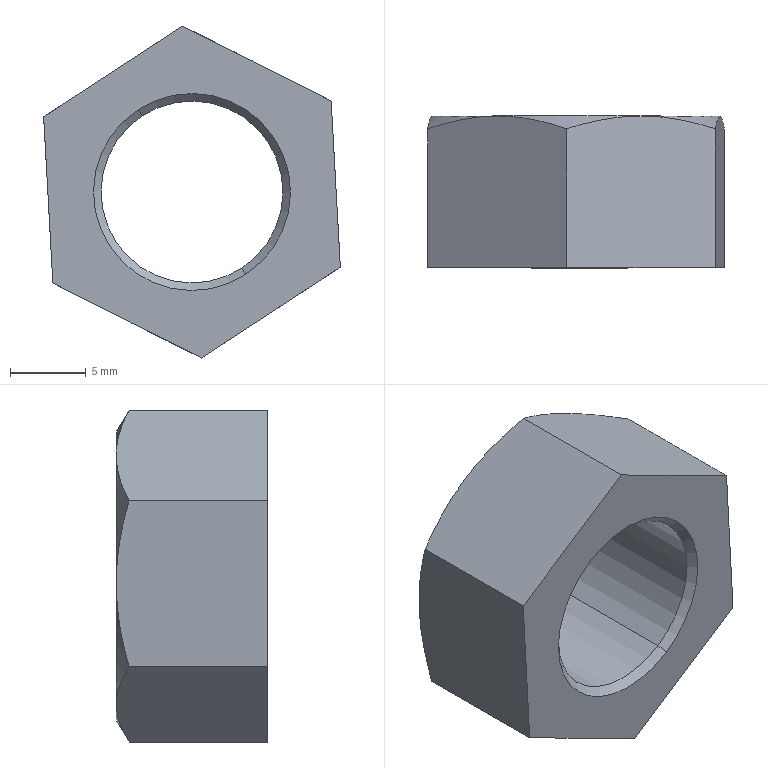Component | SolidWorks | TBK51-M12-4 | 1 solid | 20 faces | box 19.58 x 10 x 21.91 mm | volume 1978 mm3 | cone 10 | plane 8 | cylinder 2 | commonest cylinder face diameters 12 x2
STEP:
#1=CARTESIAN_POINT('',(-1.368,2.313,8.835));
#2=VERTEX_POINT('',#1);
#3=CARTESIAN_POINT('',(-1.627,2.313,9.231));
#4=VERTEX_POINT('',#3);
#5=CARTESIAN_POINT('',(-1.497,2.313,9.033));
#6=DIRECTION('',(0.,1.,-0.));
#7=DIRECTION('',(-0.5469,0.,0.8372));
#8=AXIS2_PLACEMENT_3D('',#5,#6,#7);
#9=CIRCLE('',#8,0.2362);
#10=EDGE_CURVE('',#2,#4,#9,.T.);
#11=ORIENTED_EDGE('',*,*,#10,.T.);
#12=CARTESIAN_POINT('',(-1.637,2.293,9.247));
#13=VERTEX_POINT('',#12);
#14=CARTESIAN_POINT('',(-1.627,2.313,9.231));
#15=DIRECTION('',(-0.3867,-0.7071,0.592));
#16=VECTOR('',#15,39.37);
#17=LINE('',#14,#16);
#18=EDGE_CURVE('',#4,#13,#17,.T.);
#19=ORIENTED_EDGE('',*,*,#18,.T.);
#20=CARTESIAN_POINT('',(-1.358,2.293,8.819));
#21=VERTEX_POINT('',#20);
#22=CARTESIAN_POINT('',(-1.497,2.293,9.033));
#23=DIRECTION('',(0.,1.,-0.));
#24=DIRECTION('',(-0.5469,0.,0.8372));
#25=AXIS2_PLACEMENT_3D('',#22,#23,#24);
#26=CIRCLE('',#25,0.2559);
#27=EDGE_CURVE('',#21,#13,#26,.T.);
#28=ORIENTED_EDGE('',*,*,#27,.F.);
#29=CARTESIAN_POINT('',(-1.368,2.313,8.835));
#30=DIRECTION('',(0.3867,-0.7071,-0.592));
#31=VECTOR('',#30,39.37);
#32=LINE('',#29,#31);
#33=EDGE_CURVE('',#2,#21,#32,.T.);
#34=ORIENTED_EDGE('',*,*,#33,.F.);
#35=EDGE_LOOP('',(#11,#19,#28,#34));
#36=FACE_OUTER_BOUND('',#35,.T.);
#37=CARTESIAN_POINT('',(-1.497,2.313,9.033));
#38=DIRECTION('',(-0.,-1.,0.));
#39=DIRECTION('',(0.5469,-0.,-0.8372));
#40=AXIS2_PLACEMENT_3D('',#37,#38,#39);
#41=CONICAL_SURFACE('',#40,0.2362,0.7854);
#42=ADVANCED_FACE('',(#36),#41,.F.);
#43=ORIENTED_EDGE('',*,*,#10,.F.);
#44=CARTESIAN_POINT('',(-1.368,2.667,8.835));
#45=VERTEX_POINT('',#44);
#46=CARTESIAN_POINT('',(-1.368,0.7185,8.835));
#47=DIRECTION('',(0.,1.,-0.));
#48=VECTOR('',#47,39.37);
#49=LINE('',#46,#48);
#50=EDGE_CURVE('',#2,#45,#49,.T.);
#51=ORIENTED_EDGE('',*,*,#50,.T.);
#52=CARTESIAN_POINT('',(-1.627,2.667,9.231));
#53=VERTEX_POINT('',#52);
#54=CARTESIAN_POINT('',(-1.497,2.667,9.033));
#55=DIRECTION('',(0.,1.,-0.));
#56=DIRECTION('',(-0.5469,0.,0.8372));
#57=AXIS2_PLACEMENT_3D('',#54,#55,#56);
#58=CIRCLE('',#57,0.2362);
#59=EDGE_CURVE('',#45,#53,#58,.T.);
#60=ORIENTED_EDGE('',*,*,#59,.T.);
#61=CARTESIAN_POINT('',(-1.627,0.7185,9.231));
#62=DIRECTION('',(0.,1.,-0.));
#63=VECTOR('',#62,39.37);
#64=LINE('',#61,#63);
#65=EDGE_CURVE('',#4,#53,#64,.T.);
#66=ORIENTED_EDGE('',*,*,#65,.F.);
#67=EDGE_LOOP('',(#43,#51,#60,#66));
#68=FACE_OUTER_BOUND('',#67,.T.);
#69=CARTESIAN_POINT('',(-1.497,0.7185,9.033));
#70=DIRECTION('',(0.,1.,-0.));
#71=DIRECTION('',(-0.5469,0.,0.8372));
#72=AXIS2_PLACEMENT_3D('',#69,#70,#71);
#73=CYLINDRICAL_SURFACE('',#72,0.2362);
#74=ADVANCED_FACE('',(#68),#73,.F.);
#75=ORIENTED_EDGE('',*,*,#59,.F.);
#76=CARTESIAN_POINT('',(-1.358,2.687,8.819));
#77=VERTEX_POINT('',#76);
#78=CARTESIAN_POINT('',(-1.358,2.687,8.819));
#79=DIRECTION('',(0.3867,0.7071,-0.592));
#80=VECTOR('',#79,39.37);
#81=LINE('',#78,#80);
#82=EDGE_CURVE('',#45,#77,#81,.T.);
#83=ORIENTED_EDGE('',*,*,#82,.T.);
#84=CARTESIAN_POINT('',(-1.637,2.687,9.247));
#85=VERTEX_POINT('',#84);
#86=CARTESIAN_POINT('',(-1.497,2.687,9.033));
#87=DIRECTION('',(0.,1.,-0.));
#88=DIRECTION('',(-0.5469,0.,0.8372));
#89=AXIS2_PLACEMENT_3D('',#86,#87,#88);
#90=CIRCLE('',#89,0.2559);
#91=EDGE_CURVE('',#77,#85,#90,.T.);
#92=ORIENTED_EDGE('',*,*,#91,.T.);
#93=CARTESIAN_POINT('',(-1.637,2.687,9.247));
#94=DIRECTION('',(-0.3867,0.7071,0.592));
#95=VECTOR('',#94,39.37);
#96=LINE('',#93,#95);
#97=EDGE_CURVE('',#53,#85,#96,.T.);
#98=ORIENTED_EDGE('',*,*,#97,.F.);
#99=EDGE_LOOP('',(#75,#83,#92,#98));
#100=FACE_OUTER_BOUND('',#99,.T.);
#101=CARTESIAN_POINT('',(-1.497,2.687,9.033));
#102=DIRECTION('',(0.,1.,-0.));
#103=DIRECTION('',(-0.5469,0.,0.8372));
#104=AXIS2_PLACEMENT_3D('',#101,#102,#103);
#105=CONICAL_SURFACE('',#104,0.2559,0.7854);
#106=ADVANCED_FACE('',(#100),#105,.F.);
#107=CARTESIAN_POINT('',(-1.293,2.687,8.72));
#108=VERTEX_POINT('',#107);
#109=CARTESIAN_POINT('',(-1.474,2.654,8.602));
#110=VERTEX_POINT('',#109);
#111=CARTESIAN_POINT('',(-1.293,2.687,8.72));
#112=CARTESIAN_POINT('',(-1.323,2.687,8.7));
#113=CARTESIAN_POINT('',(-1.354,2.684,8.68));
#114=CARTESIAN_POINT('',(-1.414,2.672,8.641));
#115=CARTESIAN_POINT('',(-1.444,2.664,8.621));
#116=CARTESIAN_POINT('',(-1.474,2.654,8.602));
#117=B_SPLINE_CURVE_WITH_KNOTS('',3,(#111,#112,#113,#114,#115,#116),.UNSPECIFIED.,.F.,.F.,(4,2,4),(0.02977,0.03254,0.03532),.UNSPECIFIED.);
#118=EDGE_CURVE('',#108,#110,#117,.T.);
#119=ORIENTED_EDGE('',*,*,#118,.T.);
#120=CARTESIAN_POINT('',(-1.666,2.687,8.699));
#121=VERTEX_POINT('',#120);
#122=CARTESIAN_POINT('',(-1.474,2.654,8.602));
#123=CARTESIAN_POINT('',(-1.505,2.664,8.618));
#124=CARTESIAN_POINT('',(-1.537,2.672,8.634));
#125=CARTESIAN_POINT('',(-1.601,2.684,8.666));
#126=CARTESIAN_POINT('',(-1.634,2.687,8.683));
#127=CARTESIAN_POINT('',(-1.666,2.687,8.699));
#128=B_SPLINE_CURVE_WITH_KNOTS('',3,(#122,#123,#124,#125,#126,#127),.UNSPECIFIED.,.F.,.F.,(4,2,4),(0.00000024,0.002775,0.00555),.UNSPECIFIED.);
#129=EDGE_CURVE('',#110,#121,#128,.T.);
#130=ORIENTED_EDGE('',*,*,#129,.T.);
#131=CARTESIAN_POINT('',(-1.497,2.687,9.033));
#132=DIRECTION('',(0.,1.,-0.));
#133=DIRECTION('',(-0.5469,0.,0.8372));
#134=AXIS2_PLACEMENT_3D('',#131,#132,#133);
#135=CIRCLE('',#134,0.374);
#136=EDGE_CURVE('',#108,#121,#135,.T.);
#137=ORIENTED_EDGE('',*,*,#136,.F.);
#138=EDGE_LOOP('',(#119,#130,#137));
#139=FACE_OUTER_BOUND('',#138,.T.);
#140=CARTESIAN_POINT('',(-1.497,2.631,9.033));
#141=DIRECTION('',(-0.,-1.,0.));
#142=DIRECTION('',(0.5469,-0.,-0.8372));
#143=AXIS2_PLACEMENT_3D('',#140,#141,#142);
#144=CONICAL_SURFACE('',#143,0.4705,1.047);
#145=ADVANCED_FACE('',(#139),#144,.T.);
#146=CARTESIAN_POINT('',(-1.871,2.687,9.012));
#147=VERTEX_POINT('',#146);
#148=CARTESIAN_POINT('',(-1.497,2.687,9.033));
#149=DIRECTION('',(0.,1.,-0.));
#150=DIRECTION('',(-0.5469,0.,0.8372));
#151=AXIS2_PLACEMENT_3D('',#148,#149,#150);
#152=CIRCLE('',#151,0.374);
#153=EDGE_CURVE('',#121,#147,#152,.T.);
#154=ORIENTED_EDGE('',*,*,#153,.F.);
#155=CARTESIAN_POINT('',(-1.859,2.654,8.797));
#156=VERTEX_POINT('',#155);
#157=CARTESIAN_POINT('',(-1.666,2.687,8.699));
#158=CARTESIAN_POINT('',(-1.683,2.687,8.708));
#159=CARTESIAN_POINT('',(-1.699,2.686,8.716));
#160=CARTESIAN_POINT('',(-1.732,2.683,8.732));
#161=CARTESIAN_POINT('',(-1.748,2.681,8.741));
#162=CARTESIAN_POINT('',(-1.796,2.672,8.765));
#163=CARTESIAN_POINT('',(-1.828,2.664,8.781));
#164=CARTESIAN_POINT('',(-1.859,2.654,8.797));
#165=B_SPLINE_CURVE_WITH_KNOTS('',3,(#157,#158,#159,#160,#161,#162,#163,#164),.UNSPECIFIED.,.F.,.F.,(4,2,2,4),(0.00555,0.006932,0.008314,0.01108),.UNSPECIFIED.);
#166=EDGE_CURVE('',#121,#156,#165,.T.);
#167=ORIENTED_EDGE('',*,*,#166,.T.);
#168=CARTESIAN_POINT('',(-1.859,2.654,8.797));
#169=CARTESIAN_POINT('',(-1.861,2.664,8.832));
#170=CARTESIAN_POINT('',(-1.863,2.672,8.868));
#171=CARTESIAN_POINT('',(-1.867,2.684,8.939));
#172=CARTESIAN_POINT('',(-1.869,2.687,8.976));
#173=CARTESIAN_POINT('',(-1.871,2.687,9.012));
#174=B_SPLINE_CURVE_WITH_KNOTS('',3,(#168,#169,#170,#171,#172,#173),.UNSPECIFIED.,.F.,.F.,(4,2,4),(0.00000024,0.002775,0.00555),.UNSPECIFIED.);
#175=EDGE_CURVE('',#156,#147,#174,.T.);
#176=ORIENTED_EDGE('',*,*,#175,.T.);
#177=EDGE_LOOP('',(#154,#167,#176));
#178=FACE_OUTER_BOUND('',#177,.T.);
#179=CARTESIAN_POINT('',(-1.497,2.631,9.033));
#180=DIRECTION('',(-0.,-1.,0.));
#181=DIRECTION('',(0.5469,-0.,-0.8372));
#182=AXIS2_PLACEMENT_3D('',#179,#180,#181);
#183=CONICAL_SURFACE('',#182,0.4705,1.047);
#184=ADVANCED_FACE('',(#178),#183,.T.);
#185=CARTESIAN_POINT('',(-1.702,2.687,9.346));
#186=VERTEX_POINT('',#185);
#187=CARTESIAN_POINT('',(-1.497,2.687,9.033));
#188=DIRECTION('',(0.,1.,-0.));
#189=DIRECTION('',(-0.5469,0.,0.8372));
#190=AXIS2_PLACEMENT_3D('',#187,#188,#189);
#191=CIRCLE('',#190,0.374);
#192=EDGE_CURVE('',#147,#186,#191,.T.);
#193=ORIENTED_EDGE('',*,*,#192,.F.);
#194=CARTESIAN_POINT('',(-1.883,2.654,9.228));
#195=VERTEX_POINT('',#194);
#196=CARTESIAN_POINT('',(-1.871,2.687,9.012));
#197=CARTESIAN_POINT('',(-1.872,2.687,9.031));
#198=CARTESIAN_POINT('',(-1.873,2.686,9.049));
#199=CARTESIAN_POINT('',(-1.875,2.683,9.086));
#200=CARTESIAN_POINT('',(-1.876,2.681,9.104));
#201=CARTESIAN_POINT('',(-1.879,2.672,9.157));
#202=CARTESIAN_POINT('',(-1.881,2.664,9.193));
#203=CARTESIAN_POINT('',(-1.883,2.654,9.228));
#204=B_SPLINE_CURVE_WITH_KNOTS('',3,(#196,#197,#198,#199,#200,#201,#202,#203),.UNSPECIFIED.,.F.,.F.,(4,2,2,4),(0.00555,0.006932,0.008314,0.01108),.UNSPECIFIED.);
#205=EDGE_CURVE('',#147,#195,#204,.T.);
#206=ORIENTED_EDGE('',*,*,#205,.T.);
#207=CARTESIAN_POINT('',(-1.883,2.654,9.228));
#208=CARTESIAN_POINT('',(-1.853,2.664,9.247));
#209=CARTESIAN_POINT('',(-1.823,2.672,9.267));
#210=CARTESIAN_POINT('',(-1.763,2.684,9.306));
#211=CARTESIAN_POINT('',(-1.733,2.687,9.326));
#212=CARTESIAN_POINT('',(-1.702,2.687,9.346));
#213=B_SPLINE_CURVE_WITH_KNOTS('',3,(#207,#208,#209,#210,#211,#212),.UNSPECIFIED.,.F.,.F.,(4,2,4),(0.009873,0.01265,0.01542),.UNSPECIFIED.);
#214=EDGE_CURVE('',#195,#186,#213,.T.);
#215=ORIENTED_EDGE('',*,*,#214,.T.);
#216=EDGE_LOOP('',(#193,#206,#215));
#217=FACE_OUTER_BOUND('',#216,.T.);
#218=CARTESIAN_POINT('',(-1.497,2.631,9.033));
#219=DIRECTION('',(-0.,-1.,0.));
#220=DIRECTION('',(0.5469,-0.,-0.8372));
#221=AXIS2_PLACEMENT_3D('',#218,#219,#220);
#222=CONICAL_SURFACE('',#221,0.4705,1.047);
#223=ADVANCED_FACE('',(#217),#222,.T.);
#224=CARTESIAN_POINT('',(-1.124,2.687,9.054));
#225=VERTEX_POINT('',#224);
#226=CARTESIAN_POINT('',(-1.112,2.654,8.838));
#227=VERTEX_POINT('',#226);
#228=CARTESIAN_POINT('',(-1.124,2.687,9.054));
#229=CARTESIAN_POINT('',(-1.123,2.687,9.035));
#230=CARTESIAN_POINT('',(-1.122,2.686,9.017));
#231=CARTESIAN_POINT('',(-1.12,2.683,8.981));
#232=CARTESIAN_POINT('',(-1.119,2.681,8.963));
#233=CARTESIAN_POINT('',(-1.116,2.672,8.909));
#234=CARTESIAN_POINT('',(-1.114,2.664,8.873));
#235=CARTESIAN_POINT('',(-1.112,2.654,8.838));
#236=B_SPLINE_CURVE_WITH_KNOTS('',3,(#228,#229,#230,#231,#232,#233,#234,#235),.UNSPECIFIED.,.F.,.F.,(4,2,2,4),(0.00555,0.006932,0.008314,0.01108),.UNSPECIFIED.);
#237=EDGE_CURVE('',#225,#227,#236,.T.);
#238=ORIENTED_EDGE('',*,*,#237,.T.);
#239=CARTESIAN_POINT('',(-1.112,2.654,8.838));
#240=CARTESIAN_POINT('',(-1.141,2.664,8.819));
#241=CARTESIAN_POINT('',(-1.171,2.672,8.8));
#242=CARTESIAN_POINT('',(-1.231,2.684,8.76));
#243=CARTESIAN_POINT('',(-1.262,2.687,8.74));
#244=CARTESIAN_POINT('',(-1.293,2.687,8.72));
#245=B_SPLINE_CURVE_WITH_KNOTS('',3,(#239,#240,#241,#242,#243,#244),.UNSPECIFIED.,.F.,.F.,(4,2,4),(0.02421,0.02699,0.02977),.UNSPECIFIED.);
#246=EDGE_CURVE('',#227,#108,#245,.T.);
#247=ORIENTED_EDGE('',*,*,#246,.T.);
#248=CARTESIAN_POINT('',(-1.497,2.687,9.033));
#249=DIRECTION('',(0.,1.,-0.));
#250=DIRECTION('',(-0.5469,0.,0.8372));
#251=AXIS2_PLACEMENT_3D('',#248,#249,#250);
#252=CIRCLE('',#251,0.374);
#253=EDGE_CURVE('',#225,#108,#252,.T.);
#254=ORIENTED_EDGE('',*,*,#253,.F.);
#255=EDGE_LOOP('',(#238,#247,#254));
#256=FACE_OUTER_BOUND('',#255,.T.);
#257=CARTESIAN_POINT('',(-1.497,2.631,9.033));
#258=DIRECTION('',(-0.,-1.,0.));
#259=DIRECTION('',(0.5469,-0.,-0.8372));
#260=AXIS2_PLACEMENT_3D('',#257,#258,#259);
#261=CONICAL_SURFACE('',#260,0.4705,1.047);
#262=ADVANCED_FACE('',(#256),#261,.T.);
#263=CARTESIAN_POINT('',(-1.329,2.687,9.367));
#264=VERTEX_POINT('',#263);
#265=CARTESIAN_POINT('',(-1.497,2.687,9.033));
#266=DIRECTION('',(0.,1.,-0.));
#267=DIRECTION('',(-0.5469,0.,0.8372));
#268=AXIS2_PLACEMENT_3D('',#265,#266,#267);
#269=CIRCLE('',#268,0.374);
#270=EDGE_CURVE('',#186,#264,#269,.T.);
#271=ORIENTED_EDGE('',*,*,#270,.F.);
#272=CARTESIAN_POINT('',(-1.521,2.654,9.464));
#273=VERTEX_POINT('',#272);
#274=CARTESIAN_POINT('',(-1.702,2.687,9.346));
#275=CARTESIAN_POINT('',(-1.671,2.687,9.366));
#276=CARTESIAN_POINT('',(-1.64,2.684,9.386));
#277=CARTESIAN_POINT('',(-1.58,2.672,9.426));
#278=CARTESIAN_POINT('',(-1.551,2.664,9.445));
#279=CARTESIAN_POINT('',(-1.521,2.654,9.464));
#280=B_SPLINE_CURVE_WITH_KNOTS('',3,(#274,#275,#276,#277,#278,#279),.UNSPECIFIED.,.F.,.F.,(4,2,4),(0.01542,0.0182,0.02098),.UNSPECIFIED.);
#281=EDGE_CURVE('',#186,#273,#280,.T.);
#282=ORIENTED_EDGE('',*,*,#281,.T.);
#283=CARTESIAN_POINT('',(-1.521,2.654,9.464));
#284=CARTESIAN_POINT('',(-1.49,2.664,9.448));
#285=CARTESIAN_POINT('',(-1.458,2.672,9.432));
#286=CARTESIAN_POINT('',(-1.394,2.684,9.4));
#287=CARTESIAN_POINT('',(-1.361,2.687,9.383));
#288=CARTESIAN_POINT('',(-1.329,2.687,9.367));
#289=B_SPLINE_CURVE_WITH_KNOTS('',3,(#283,#284,#285,#286,#287,#288),.UNSPECIFIED.,.F.,.F.,(4,2,4),(0.00000024,0.002775,0.00555),.UNSPECIFIED.);
#290=EDGE_CURVE('',#273,#264,#289,.T.);
#291=ORIENTED_EDGE('',*,*,#290,.T.);
#292=EDGE_LOOP('',(#271,#282,#291));
#293=FACE_OUTER_BOUND('',#292,.T.);
#294=CARTESIAN_POINT('',(-1.497,2.631,9.033));
#295=DIRECTION('',(-0.,-1.,0.));
#296=DIRECTION('',(0.5469,-0.,-0.8372));
#297=AXIS2_PLACEMENT_3D('',#294,#295,#296);
#298=CONICAL_SURFACE('',#297,0.4705,1.047);
#299=ADVANCED_FACE('',(#293),#298,.T.);
#300=CARTESIAN_POINT('',(-1.497,2.687,9.033));
#301=DIRECTION('',(0.,1.,-0.));
#302=DIRECTION('',(-0.5469,0.,0.8372));
#303=AXIS2_PLACEMENT_3D('',#300,#301,#302);
#304=CIRCLE('',#303,0.2559);
#305=EDGE_CURVE('',#85,#77,#304,.T.);
#306=ORIENTED_EDGE('',*,*,#305,.F.);
#307=ORIENTED_EDGE('',*,*,#91,.F.);
#308=EDGE_LOOP('',(#306,#307));
#309=FACE_BOUND('',#308,.T.);
#310=ORIENTED_EDGE('',*,*,#270,.T.);
#311=CARTESIAN_POINT('',(-1.497,2.687,9.033));
#312=DIRECTION('',(0.,1.,-0.));
#313=DIRECTION('',(-0.5469,0.,0.8372));
#314=AXIS2_PLACEMENT_3D('',#311,#312,#313);
#315=CIRCLE('',#314,0.374);
#316=EDGE_CURVE('',#264,#225,#315,.T.);
#317=ORIENTED_EDGE('',*,*,#316,.T.);
#318=ORIENTED_EDGE('',*,*,#253,.T.);
#319=ORIENTED_EDGE('',*,*,#136,.T.);
#320=ORIENTED_EDGE('',*,*,#153,.T.);
#321=ORIENTED_EDGE('',*,*,#192,.T.);
#322=EDGE_LOOP('',(#310,#317,#318,#319,#320,#321));
#323=FACE_OUTER_BOUND('',#322,.T.);
#324=CARTESIAN_POINT('',(-1.184,2.687,9.238));
#325=DIRECTION('',(-0.,-1.,0.));
#326=DIRECTION('',(0.5469,-0.,-0.8372));
#327=AXIS2_PLACEMENT_3D('',#324,#325,#326);
#328=PLANE('',#327);
#329=ADVANCED_FACE('',(#309,#323),#328,.F.);
#330=ORIENTED_EDGE('',*,*,#82,.F.);
#331=CARTESIAN_POINT('',(-1.497,2.667,9.033));
#332=DIRECTION('',(0.,1.,-0.));
#333=DIRECTION('',(-0.5469,0.,0.8372));
#334=AXIS2_PLACEMENT_3D('',#331,#332,#333);
#335=CIRCLE('',#334,0.2362);
#336=EDGE_CURVE('',#53,#45,#335,.T.);
#337=ORIENTED_EDGE('',*,*,#336,.F.);
#338=ORIENTED_EDGE('',*,*,#97,.T.);
#339=ORIENTED_EDGE('',*,*,#305,.T.);
#340=EDGE_LOOP('',(#330,#337,#338,#339));
#341=FACE_OUTER_BOUND('',#340,.T.);
#342=CARTESIAN_POINT('',(-1.497,2.687,9.033));
#343=DIRECTION('',(0.,1.,-0.));
#344=DIRECTION('',(-0.5469,0.,0.8372));
#345=AXIS2_PLACEMENT_3D('',#342,#343,#344);
#346=CONICAL_SURFACE('',#345,0.2559,0.7854);
#347=ADVANCED_FACE('',(#341),#346,.F.);
#348=ORIENTED_EDGE('',*,*,#50,.F.);
#349=CARTESIAN_POINT('',(-1.497,2.313,9.033));
#350=DIRECTION('',(0.,1.,-0.));
#351=DIRECTION('',(-0.5469,0.,0.8372));
#352=AXIS2_PLACEMENT_3D('',#349,#350,#351);
#353=CIRCLE('',#352,0.2362);
#354=EDGE_CURVE('',#4,#2,#353,.T.);
#355=ORIENTED_EDGE('',*,*,#354,.F.);
#356=ORIENTED_EDGE('',*,*,#65,.T.);
#357=ORIENTED_EDGE('',*,*,#336,.T.);
#358=EDGE_LOOP('',(#348,#355,#356,#357));
#359=FACE_OUTER_BOUND('',#358,.T.);
#360=CARTESIAN_POINT('',(-1.497,0.7185,9.033));
#361=DIRECTION('',(0.,1.,-0.));
#362=DIRECTION('',(-0.5469,0.,0.8372));
#363=AXIS2_PLACEMENT_3D('',#360,#361,#362);
#364=CYLINDRICAL_SURFACE('',#363,0.2362);
#365=ADVANCED_FACE('',(#359),#364,.F.);
#366=ORIENTED_EDGE('',*,*,#18,.F.);
#367=ORIENTED_EDGE('',*,*,#354,.T.);
#368=ORIENTED_EDGE('',*,*,#33,.T.);
#369=CARTESIAN_POINT('',(-1.497,2.293,9.033));
#370=DIRECTION('',(0.,1.,-0.));
#371=DIRECTION('',(-0.5469,0.,0.8372));
#372=AXIS2_PLACEMENT_3D('',#369,#370,#371);
#373=CIRCLE('',#372,0.2559);
#374=EDGE_CURVE('',#13,#21,#373,.T.);
#375=ORIENTED_EDGE('',*,*,#374,.F.);
#376=EDGE_LOOP('',(#366,#367,#368,#375));
#377=FACE_OUTER_BOUND('',#376,.T.);
#378=CARTESIAN_POINT('',(-1.497,2.313,9.033));
#379=DIRECTION('',(-0.,-1.,0.));
#380=DIRECTION('',(0.5469,-0.,-0.8372));
#381=AXIS2_PLACEMENT_3D('',#378,#379,#380);
#382=CONICAL_SURFACE('',#381,0.2362,0.7854);
#383=ADVANCED_FACE('',(#377),#382,.F.);
#384=CARTESIAN_POINT('',(-1.136,2.293,9.269));
#385=VERTEX_POINT('',#384);
#386=CARTESIAN_POINT('',(-1.521,2.293,9.464));
#387=VERTEX_POINT('',#386);
#388=CARTESIAN_POINT('',(-1.136,2.293,9.269));
#389=DIRECTION('',(-0.8923,0.,0.4515));
#390=VECTOR('',#389,39.37);
#391=LINE('',#388,#390);
#392=EDGE_CURVE('',#385,#387,#391,.T.);
#393=ORIENTED_EDGE('',*,*,#392,.T.);
#394=CARTESIAN_POINT('',(-1.883,2.293,9.228));
#395=VERTEX_POINT('',#394);
#396=CARTESIAN_POINT('',(-1.521,2.293,9.464));
#397=DIRECTION('',(-0.8372,0.,-0.5469));
#398=VECTOR('',#397,39.37);
#399=LINE('',#396,#398);
#400=EDGE_CURVE('',#387,#395,#399,.T.);
#401=ORIENTED_EDGE('',*,*,#400,.T.);
#402=CARTESIAN_POINT('',(-1.859,2.293,8.797));
#403=VERTEX_POINT('',#402);
#404=CARTESIAN_POINT('',(-1.883,2.293,9.228));
#405=DIRECTION('',(0.05508,-0.,-0.9985));
#406=VECTOR('',#405,39.37);
#407=LINE('',#404,#406);
#408=EDGE_CURVE('',#395,#403,#407,.T.);
#409=ORIENTED_EDGE('',*,*,#408,.T.);
#410=CARTESIAN_POINT('',(-1.474,2.293,8.602));
#411=VERTEX_POINT('',#410);
#412=CARTESIAN_POINT('',(-1.859,2.293,8.797));
#413=DIRECTION('',(0.8923,-0.,-0.4515));
#414=VECTOR('',#413,39.37);
#415=LINE('',#412,#414);
#416=EDGE_CURVE('',#403,#411,#415,.T.);
#417=ORIENTED_EDGE('',*,*,#416,.T.);
#418=CARTESIAN_POINT('',(-1.112,2.293,8.838));
#419=VERTEX_POINT('',#418);
#420=CARTESIAN_POINT('',(-1.474,2.293,8.602));
#421=DIRECTION('',(0.8372,-0.,0.5469));
#422=VECTOR('',#421,39.37);
#423=LINE('',#420,#422);
#424=EDGE_CURVE('',#411,#419,#423,.T.);
#425=ORIENTED_EDGE('',*,*,#424,.T.);
#426=CARTESIAN_POINT('',(-1.112,2.293,8.838));
#427=DIRECTION('',(-0.05508,0.,0.9985));
#428=VECTOR('',#427,39.37);
#429=LINE('',#426,#428);
#430=EDGE_CURVE('',#419,#385,#429,.T.);
#431=ORIENTED_EDGE('',*,*,#430,.T.);
#432=EDGE_LOOP('',(#393,#401,#409,#417,#425,#431));
#433=FACE_OUTER_BOUND('',#432,.T.);
#434=ORIENTED_EDGE('',*,*,#27,.T.);
#435=ORIENTED_EDGE('',*,*,#374,.T.);
#436=EDGE_LOOP('',(#434,#435));
#437=FACE_BOUND('',#436,.T.);
#438=CARTESIAN_POINT('',(-1.283,2.293,9.173));
#439=DIRECTION('',(0.,1.,-0.));
#440=DIRECTION('',(-0.5469,0.,0.8372));
#441=AXIS2_PLACEMENT_3D('',#438,#439,#440);
#442=PLANE('',#441);
#443=ADVANCED_FACE('',(#433,#437),#442,.F.);
#444=CARTESIAN_POINT('',(-1.136,2.654,9.269));
#445=VERTEX_POINT('',#444);
#446=CARTESIAN_POINT('',(-1.329,2.687,9.367));
#447=CARTESIAN_POINT('',(-1.312,2.687,9.359));
#448=CARTESIAN_POINT('',(-1.296,2.686,9.35));
#449=CARTESIAN_POINT('',(-1.263,2.683,9.334));
#450=CARTESIAN_POINT('',(-1.247,2.681,9.326));
#451=CARTESIAN_POINT('',(-1.199,2.672,9.301));
#452=CARTESIAN_POINT('',(-1.167,2.664,9.285));
#453=CARTESIAN_POINT('',(-1.136,2.654,9.269));
#454=B_SPLINE_CURVE_WITH_KNOTS('',3,(#446,#447,#448,#449,#450,#451,#452,#453),.UNSPECIFIED.,.F.,.F.,(4,2,2,4),(0.00555,0.006932,0.008314,0.01108),.UNSPECIFIED.);
#455=EDGE_CURVE('',#264,#445,#454,.T.);
#456=ORIENTED_EDGE('',*,*,#455,.T.);
#457=CARTESIAN_POINT('',(-1.136,2.654,9.269));
#458=CARTESIAN_POINT('',(-1.134,2.664,9.234));
#459=CARTESIAN_POINT('',(-1.132,2.672,9.198));
#460=CARTESIAN_POINT('',(-1.128,2.684,9.127));
#461=CARTESIAN_POINT('',(-1.126,2.687,9.09));
#462=CARTESIAN_POINT('',(-1.124,2.687,9.054));
#463=B_SPLINE_CURVE_WITH_KNOTS('',3,(#457,#458,#459,#460,#461,#462),.UNSPECIFIED.,.F.,.F.,(4,2,4),(0.00000024,0.002775,0.00555),.UNSPECIFIED.);
#464=EDGE_CURVE('',#445,#225,#463,.T.);
#465=ORIENTED_EDGE('',*,*,#464,.T.);
#466=ORIENTED_EDGE('',*,*,#316,.F.);
#467=EDGE_LOOP('',(#456,#465,#466));
#468=FACE_OUTER_BOUND('',#467,.T.);
#469=CARTESIAN_POINT('',(-1.497,2.631,9.033));
#470=DIRECTION('',(-0.,-1.,0.));
#471=DIRECTION('',(0.5469,-0.,-0.8372));
#472=AXIS2_PLACEMENT_3D('',#469,#470,#471);
#473=CONICAL_SURFACE('',#472,0.4705,1.047);
#474=ADVANCED_FACE('',(#468),#473,.T.);
#475=CARTESIAN_POINT('',(-1.883,2.293,9.228));
#476=DIRECTION('',(0.,1.,-0.));
#477=VECTOR('',#476,39.37);
#478=LINE('',#475,#477);
#479=EDGE_CURVE('',#395,#195,#478,.T.);
#480=ORIENTED_EDGE('',*,*,#479,.F.);
#481=ORIENTED_EDGE('',*,*,#400,.F.);
#482=CARTESIAN_POINT('',(-1.521,2.293,9.464));
#483=DIRECTION('',(0.,1.,-0.));
#484=VECTOR('',#483,39.37);
#485=LINE('',#482,#484);
#486=EDGE_CURVE('',#387,#273,#485,.T.);
#487=ORIENTED_EDGE('',*,*,#486,.T.);
#488=ORIENTED_EDGE('',*,*,#281,.F.);
#489=ORIENTED_EDGE('',*,*,#214,.F.);
#490=EDGE_LOOP('',(#480,#481,#487,#488,#489));
#491=FACE_OUTER_BOUND('',#490,.T.);
#492=CARTESIAN_POINT('',(-1.521,2.293,9.464));
#493=DIRECTION('',(0.5469,-0.,-0.8372));
#494=DIRECTION('',(0.,1.,-0.));
#495=AXIS2_PLACEMENT_3D('',#492,#493,#494);
#496=PLANE('',#495);
#497=ADVANCED_FACE('',(#491),#496,.F.);
#498=CARTESIAN_POINT('',(-1.859,2.293,8.797));
#499=DIRECTION('',(0.,1.,-0.));
#500=VECTOR('',#499,39.37);
#501=LINE('',#498,#500);
#502=EDGE_CURVE('',#403,#156,#501,.T.);
#503=ORIENTED_EDGE('',*,*,#502,.F.);
#504=ORIENTED_EDGE('',*,*,#408,.F.);
#505=ORIENTED_EDGE('',*,*,#479,.T.);
#506=ORIENTED_EDGE('',*,*,#205,.F.);
#507=ORIENTED_EDGE('',*,*,#175,.F.);
#508=EDGE_LOOP('',(#503,#504,#505,#506,#507));
#509=FACE_OUTER_BOUND('',#508,.T.);
#510=CARTESIAN_POINT('',(-1.883,2.293,9.228));
#511=DIRECTION('',(0.9985,-0.,0.05508));
#512=DIRECTION('',(-0.05508,0.,0.9985));
#513=AXIS2_PLACEMENT_3D('',#510,#511,#512);
#514=PLANE('',#513);
#515=ADVANCED_FACE('',(#509),#514,.F.);
#516=CARTESIAN_POINT('',(-1.474,2.293,8.602));
#517=DIRECTION('',(0.,1.,-0.));
#518=VECTOR('',#517,39.37);
#519=LINE('',#516,#518);
#520=EDGE_CURVE('',#411,#110,#519,.T.);
#521=ORIENTED_EDGE('',*,*,#520,.F.);
#522=ORIENTED_EDGE('',*,*,#416,.F.);
#523=ORIENTED_EDGE('',*,*,#502,.T.);
#524=ORIENTED_EDGE('',*,*,#166,.F.);
#525=ORIENTED_EDGE('',*,*,#129,.F.);
#526=EDGE_LOOP('',(#521,#522,#523,#524,#525));
#527=FACE_OUTER_BOUND('',#526,.T.);
#528=CARTESIAN_POINT('',(-1.859,2.293,8.797));
#529=DIRECTION('',(0.4515,-0.,0.8923));
#530=DIRECTION('',(-0.8923,0.,0.4515));
#531=AXIS2_PLACEMENT_3D('',#528,#529,#530);
#532=PLANE('',#531);
#533=ADVANCED_FACE('',(#527),#532,.F.);
#534=CARTESIAN_POINT('',(-1.112,2.293,8.838));
#535=DIRECTION('',(0.,1.,-0.));
#536=VECTOR('',#535,39.37);
#537=LINE('',#534,#536);
#538=EDGE_CURVE('',#419,#227,#537,.T.);
#539=ORIENTED_EDGE('',*,*,#538,.F.);
#540=ORIENTED_EDGE('',*,*,#424,.F.);
#541=ORIENTED_EDGE('',*,*,#520,.T.);
#542=ORIENTED_EDGE('',*,*,#118,.F.);
#543=ORIENTED_EDGE('',*,*,#246,.F.);
#544=EDGE_LOOP('',(#539,#540,#541,#542,#543));
#545=FACE_OUTER_BOUND('',#544,.T.);
#546=CARTESIAN_POINT('',(-1.474,2.293,8.602));
#547=DIRECTION('',(-0.5469,0.,0.8372));
#548=DIRECTION('',(-0.,-1.,0.));
#549=AXIS2_PLACEMENT_3D('',#546,#547,#548);
#550=PLANE('',#549);
#551=ADVANCED_FACE('',(#545),#550,.F.);
#552=CARTESIAN_POINT('',(-1.136,2.293,9.269));
#553=DIRECTION('',(0.,1.,-0.));
#554=VECTOR('',#553,39.37);
#555=LINE('',#552,#554);
#556=EDGE_CURVE('',#385,#445,#555,.T.);
#557=ORIENTED_EDGE('',*,*,#556,.F.);
#558=ORIENTED_EDGE('',*,*,#430,.F.);
#559=ORIENTED_EDGE('',*,*,#538,.T.);
#560=ORIENTED_EDGE('',*,*,#237,.F.);
#561=ORIENTED_EDGE('',*,*,#464,.F.);
#562=EDGE_LOOP('',(#557,#558,#559,#560,#561));
#563=FACE_OUTER_BOUND('',#562,.T.);
#564=CARTESIAN_POINT('',(-1.112,2.293,8.838));
#565=DIRECTION('',(-0.9985,0.,-0.05508));
#566=DIRECTION('',(0.05508,-0.,-0.9985));
#567=AXIS2_PLACEMENT_3D('',#564,#565,#566);
#568=PLANE('',#567);
#569=ADVANCED_FACE('',(#563),#568,.F.);
#570=ORIENTED_EDGE('',*,*,#486,.F.);
#571=ORIENTED_EDGE('',*,*,#392,.F.);
#572=ORIENTED_EDGE('',*,*,#556,.T.);
#573=ORIENTED_EDGE('',*,*,#455,.F.);
#574=ORIENTED_EDGE('',*,*,#290,.F.);
#575=EDGE_LOOP('',(#570,#571,#572,#573,#574));
#576=FACE_OUTER_BOUND('',#575,.T.);
#577=CARTESIAN_POINT('',(-1.136,2.293,9.269));
#578=DIRECTION('',(-0.4515,0.,-0.8923));
#579=DIRECTION('',(0.8923,-0.,-0.4515));
#580=AXIS2_PLACEMENT_3D('',#577,#578,#579);
#581=PLANE('',#580);
#582=ADVANCED_FACE('',(#576),#581,.F.);
#583=CLOSED_SHELL('',(#42,#74,#106,#145,#184,#223,#262,#299,#329,#347,#365,#383,#443,#474,#497,#515,#533,#551,#569,#582));
#584=MANIFOLD_SOLID_BREP('',#583);
#585=CARTESIAN_POINT('',(0.,0.,0.));
#586=DIRECTION('',(0.,0.,1.));
#587=DIRECTION('',(1.,0.,0.));
#588=AXIS2_PLACEMENT_3D('',#585,#586,#587);
#589=(LENGTH_UNIT()NAMED_UNIT(*)SI_UNIT($,.METRE.));
#590=LENGTH_MEASURE_WITH_UNIT(LENGTH_MEASURE(0.0254),#589);
#591=DIMENSIONAL_EXPONENTS(1.,0.,0.,0.,0.,0.,0.);
#592=(CONVERSION_BASED_UNIT('',#590)LENGTH_UNIT()NAMED_UNIT(#591));
#593=UNCERTAINTY_MEASURE_WITH_UNIT(LENGTH_MEASURE(0.00001),#592,'','');
#594=(NAMED_UNIT(*)PLANE_ANGLE_UNIT()SI_UNIT($,.RADIAN.));
#595=(NAMED_UNIT(*)SI_UNIT($,.STERADIAN.)SOLID_ANGLE_UNIT());
#596=(GEOMETRIC_REPRESENTATION_CONTEXT(3)GLOBAL_UNCERTAINTY_ASSIGNED_CONTEXT((#593))GLOBAL_UNIT_ASSIGNED_CONTEXT((#592,#594,#595))REPRESENTATION_CONTEXT('',''));
#597=ADVANCED_BREP_SHAPE_REPRESENTATION('',(#584,#588),#596);
#598=COLOUR_RGB('',0.7922,0.8196,0.9333);
#599=FILL_AREA_STYLE_COLOUR('',#598);
#600=FILL_AREA_STYLE('',(#599));
#601=SURFACE_STYLE_FILL_AREA(#600);
#602=SURFACE_SIDE_STYLE('',(#601));
#603=SURFACE_STYLE_USAGE(.BOTH.,#602);
#604=PRESENTATION_STYLE_ASSIGNMENT((#603));
#605=STYLED_ITEM('',(#604),#584);
#606=PRESENTATION_LAYER_ASSIGNMENT('','',(#605));
#607=(LENGTH_UNIT()NAMED_UNIT(*)SI_UNIT($,.METRE.));
#608=LENGTH_MEASURE_WITH_UNIT(LENGTH_MEASURE(0.0254),#607);
#609=DIMENSIONAL_EXPONENTS(1.,0.,0.,0.,0.,0.,0.);
#610=(CONVERSION_BASED_UNIT('',#608)LENGTH_UNIT()NAMED_UNIT(#609));
#611=UNCERTAINTY_MEASURE_WITH_UNIT(LENGTH_MEASURE(0.00001),#610,'','');
#612=(NAMED_UNIT(*)PLANE_ANGLE_UNIT()SI_UNIT($,.RADIAN.));
#613=(NAMED_UNIT(*)SI_UNIT($,.STERADIAN.)SOLID_ANGLE_UNIT());
#614=(GEOMETRIC_REPRESENTATION_CONTEXT(3)GLOBAL_UNCERTAINTY_ASSIGNED_CONTEXT((#611))GLOBAL_UNIT_ASSIGNED_CONTEXT((#610,#612,#613))REPRESENTATION_CONTEXT('',''));
#615=MECHANICAL_DESIGN_GEOMETRIC_PRESENTATION_REPRESENTATION('',(#605),#614);